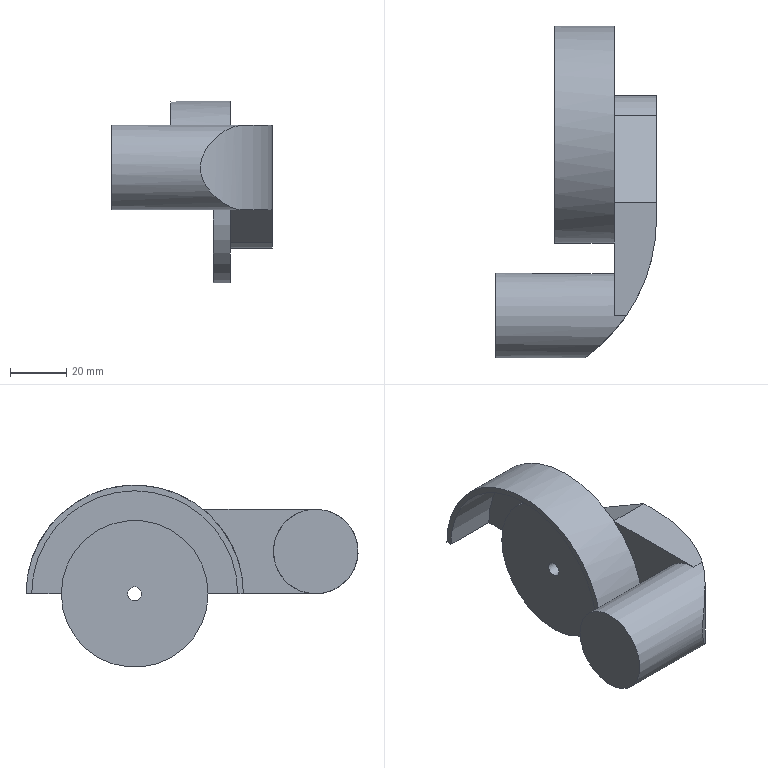Component | NX | WHEEL_BRACKET | 1 solid | 19 faces | volume 79112 mm3 | plane 12 | cylinder 7 | commonest cylinder face diameters 5 x1 52 x1 27.586 x1 30 x1 77 x1 73 x1 120 x1